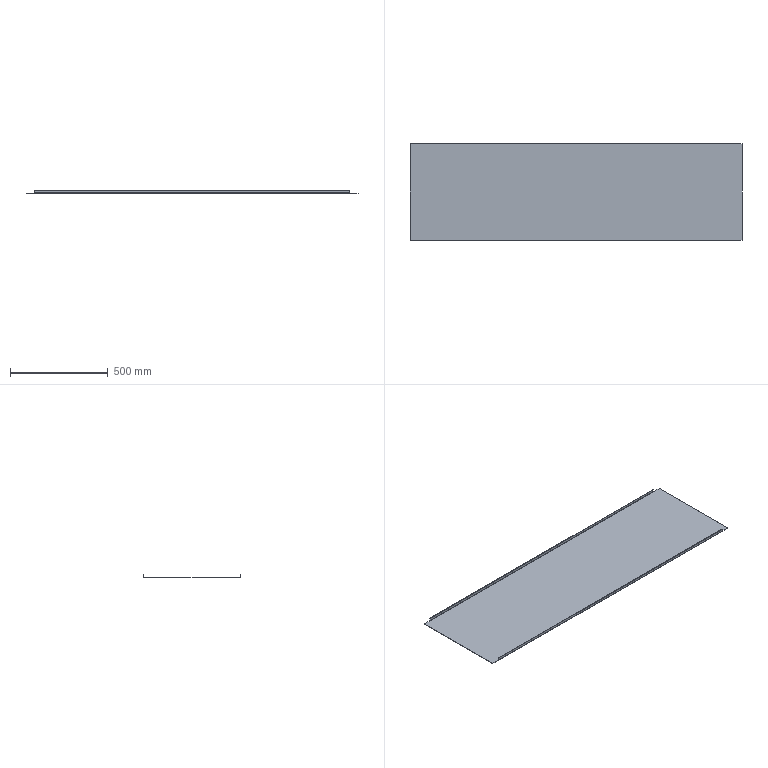Component | SolidWorks | RearBackPlate-1 | 1 solid | 22 faces | box 1700 x 500 x 15 mm | volume 1777475 mm3 | plane 18 | cylinder 4 | commonest cylinder face diameters 6 x2 2 x2
STEP:
#1=COLOUR_RGB('',0.7922,0.8196,0.9333);
#2=FILL_AREA_STYLE_COLOUR('',#1);
#3=FILL_AREA_STYLE('',(#2));
#4=SURFACE_STYLE_FILL_AREA(#3);
#5=SURFACE_SIDE_STYLE('',(#4));
#6=SURFACE_STYLE_USAGE(.BOTH.,#5);
#7=PRESENTATION_STYLE_ASSIGNMENT((#6));
#8=CARTESIAN_POINT('',(28.746,-4.158,0.03937));
#9=VERTEX_POINT('',#8);
#10=CARTESIAN_POINT('',(-34.876,-4.158,0.03937));
#11=VERTEX_POINT('',#10);
#12=CARTESIAN_POINT('',(-36.529,-4.158,0.03937));
#13=DIRECTION('',(-1.,0.,0.));
#14=VECTOR('',#13,39.37);
#15=LINE('',#12,#14);
#16=EDGE_CURVE('',#9,#11,#15,.T.);
#17=ORIENTED_EDGE('',*,*,#16,.T.);
#18=CARTESIAN_POINT('',(-34.876,-4.04,-0.07874));
#19=VERTEX_POINT('',#18);
#20=CARTESIAN_POINT('',(-34.876,-4.04,0.03937));
#21=DIRECTION('',(1.,0.,0.));
#22=DIRECTION('',(0.,0.,1.));
#23=AXIS2_PLACEMENT_3D('',#20,#21,#22);
#24=CIRCLE('',#23,0.1181);
#25=EDGE_CURVE('',#11,#19,#24,.T.);
#26=ORIENTED_EDGE('',*,*,#25,.T.);
#27=CARTESIAN_POINT('',(28.746,-4.04,-0.07874));
#28=VERTEX_POINT('',#27);
#29=CARTESIAN_POINT('',(30.4,-4.04,-0.07874));
#30=DIRECTION('',(-1.,0.,0.));
#31=VECTOR('',#30,39.37);
#32=LINE('',#29,#31);
#33=EDGE_CURVE('',#28,#19,#32,.T.);
#34=ORIENTED_EDGE('',*,*,#33,.F.);
#35=CARTESIAN_POINT('',(28.746,-4.04,0.03937));
#36=DIRECTION('',(1.,0.,0.));
#37=DIRECTION('',(0.,0.,1.));
#38=AXIS2_PLACEMENT_3D('',#35,#36,#37);
#39=CIRCLE('',#38,0.1181);
#40=EDGE_CURVE('',#9,#28,#39,.T.);
#41=ORIENTED_EDGE('',*,*,#40,.F.);
#42=EDGE_LOOP('',(#17,#26,#34,#41));
#43=FACE_OUTER_BOUND('',#42,.T.);
#44=CARTESIAN_POINT('',(30.4,-4.04,0.03937));
#45=DIRECTION('',(1.,0.,0.));
#46=DIRECTION('',(0.,-1.,-0.));
#47=AXIS2_PLACEMENT_3D('',#44,#45,#46);
#48=CYLINDRICAL_SURFACE('',#47,0.1181);
#49=ADVANCED_FACE('',(#43),#48,.T.);
#50=CARTESIAN_POINT('',(-34.876,-4.079,0.03937));
#51=VERTEX_POINT('',#50);
#52=CARTESIAN_POINT('',(-34.876,-4.04,-0.));
#53=VERTEX_POINT('',#52);
#54=CARTESIAN_POINT('',(-34.876,-4.04,0.03937));
#55=DIRECTION('',(1.,0.,0.));
#56=DIRECTION('',(0.,0.,1.));
#57=AXIS2_PLACEMENT_3D('',#54,#55,#56);
#58=CIRCLE('',#57,0.03937);
#59=EDGE_CURVE('',#51,#53,#58,.T.);
#60=ORIENTED_EDGE('',*,*,#59,.F.);
#61=CARTESIAN_POINT('',(28.746,-4.079,0.03937));
#62=VERTEX_POINT('',#61);
#63=CARTESIAN_POINT('',(-36.529,-4.079,0.03937));
#64=DIRECTION('',(1.,0.,0.));
#65=VECTOR('',#64,39.37);
#66=LINE('',#63,#65);
#67=EDGE_CURVE('',#51,#62,#66,.T.);
#68=ORIENTED_EDGE('',*,*,#67,.T.);
#69=CARTESIAN_POINT('',(28.746,-4.04,-0.));
#70=VERTEX_POINT('',#69);
#71=CARTESIAN_POINT('',(28.746,-4.04,0.03937));
#72=DIRECTION('',(1.,0.,0.));
#73=DIRECTION('',(0.,0.,1.));
#74=AXIS2_PLACEMENT_3D('',#71,#72,#73);
#75=CIRCLE('',#74,0.03937);
#76=EDGE_CURVE('',#62,#70,#75,.T.);
#77=ORIENTED_EDGE('',*,*,#76,.T.);
#78=CARTESIAN_POINT('',(30.4,-4.04,-0.));
#79=DIRECTION('',(-1.,0.,0.));
#80=VECTOR('',#79,39.37);
#81=LINE('',#78,#80);
#82=EDGE_CURVE('',#70,#53,#81,.T.);
#83=ORIENTED_EDGE('',*,*,#82,.T.);
#84=EDGE_LOOP('',(#60,#68,#77,#83));
#85=FACE_OUTER_BOUND('',#84,.T.);
#86=CARTESIAN_POINT('',(30.4,-4.04,0.03937));
#87=DIRECTION('',(1.,0.,0.));
#88=DIRECTION('',(0.,-1.,-0.));
#89=AXIS2_PLACEMENT_3D('',#86,#87,#88);
#90=CYLINDRICAL_SURFACE('',#89,0.03937);
#91=ADVANCED_FACE('',(#85),#90,.F.);
#92=CARTESIAN_POINT('',(-34.876,-4.158,0.5118));
#93=VERTEX_POINT('',#92);
#94=CARTESIAN_POINT('',(-34.876,-4.158,-0.07874));
#95=DIRECTION('',(0.,0.,1.));
#96=VECTOR('',#95,39.37);
#97=LINE('',#94,#96);
#98=EDGE_CURVE('',#11,#93,#97,.T.);
#99=ORIENTED_EDGE('',*,*,#98,.F.);
#100=ORIENTED_EDGE('',*,*,#16,.F.);
#101=CARTESIAN_POINT('',(28.746,-4.158,0.5118));
#102=VERTEX_POINT('',#101);
#103=CARTESIAN_POINT('',(28.746,-4.158,-0.07874));
#104=DIRECTION('',(0.,0.,-1.));
#105=VECTOR('',#104,39.37);
#106=LINE('',#103,#105);
#107=EDGE_CURVE('',#102,#9,#106,.T.);
#108=ORIENTED_EDGE('',*,*,#107,.F.);
#109=CARTESIAN_POINT('',(-36.529,-4.158,0.5118));
#110=DIRECTION('',(-1.,0.,0.));
#111=VECTOR('',#110,39.37);
#112=LINE('',#109,#111);
#113=EDGE_CURVE('',#102,#93,#112,.T.);
#114=ORIENTED_EDGE('',*,*,#113,.T.);
#115=EDGE_LOOP('',(#99,#100,#108,#114));
#116=FACE_OUTER_BOUND('',#115,.T.);
#117=CARTESIAN_POINT('',(-36.529,-4.158,0.5118));
#118=DIRECTION('',(0.,1.,0.));
#119=DIRECTION('',(0.,-0.,1.));
#120=AXIS2_PLACEMENT_3D('',#117,#118,#119);
#121=PLANE('',#120);
#122=ADVANCED_FACE('',(#116),#121,.F.);
#123=ORIENTED_EDGE('',*,*,#67,.F.);
#124=CARTESIAN_POINT('',(-34.876,-4.079,0.5118));
#125=VERTEX_POINT('',#124);
#126=CARTESIAN_POINT('',(-34.876,-4.079,0.5118));
#127=DIRECTION('',(0.,-0.,1.));
#128=VECTOR('',#127,39.37);
#129=LINE('',#126,#128);
#130=EDGE_CURVE('',#51,#125,#129,.T.);
#131=ORIENTED_EDGE('',*,*,#130,.T.);
#132=CARTESIAN_POINT('',(28.746,-4.079,0.5118));
#133=VERTEX_POINT('',#132);
#134=CARTESIAN_POINT('',(-36.529,-4.079,0.5118));
#135=DIRECTION('',(-1.,0.,0.));
#136=VECTOR('',#135,39.37);
#137=LINE('',#134,#136);
#138=EDGE_CURVE('',#133,#125,#137,.T.);
#139=ORIENTED_EDGE('',*,*,#138,.F.);
#140=CARTESIAN_POINT('',(28.746,-4.079,0.5118));
#141=DIRECTION('',(0.,-0.,1.));
#142=VECTOR('',#141,39.37);
#143=LINE('',#140,#142);
#144=EDGE_CURVE('',#62,#133,#143,.T.);
#145=ORIENTED_EDGE('',*,*,#144,.F.);
#146=EDGE_LOOP('',(#123,#131,#139,#145));
#147=FACE_OUTER_BOUND('',#146,.T.);
#148=CARTESIAN_POINT('',(-36.529,-4.079,0.5118));
#149=DIRECTION('',(0.,1.,0.));
#150=DIRECTION('',(0.,-0.,1.));
#151=AXIS2_PLACEMENT_3D('',#148,#149,#150);
#152=PLANE('',#151);
#153=ADVANCED_FACE('',(#147),#152,.T.);
#154=CARTESIAN_POINT('',(-34.876,-4.04,0.5118));
#155=DIRECTION('',(0.,1.,0.));
#156=VECTOR('',#155,39.37);
#157=LINE('',#154,#156);
#158=EDGE_CURVE('',#93,#125,#157,.T.);
#159=ORIENTED_EDGE('',*,*,#158,.F.);
#160=ORIENTED_EDGE('',*,*,#113,.F.);
#161=CARTESIAN_POINT('',(28.746,-4.158,0.5118));
#162=DIRECTION('',(0.,1.,0.));
#163=VECTOR('',#162,39.37);
#164=LINE('',#161,#163);
#165=EDGE_CURVE('',#102,#133,#164,.T.);
#166=ORIENTED_EDGE('',*,*,#165,.T.);
#167=ORIENTED_EDGE('',*,*,#138,.T.);
#168=EDGE_LOOP('',(#159,#160,#166,#167));
#169=FACE_OUTER_BOUND('',#168,.T.);
#170=CARTESIAN_POINT('',(-36.529,-4.158,0.5118));
#171=DIRECTION('',(0.,0.,-1.));
#172=DIRECTION('',(0.,1.,0.));
#173=AXIS2_PLACEMENT_3D('',#170,#171,#172);
#174=PLANE('',#173);
#175=ADVANCED_FACE('',(#169),#174,.F.);
#176=CARTESIAN_POINT('',(-34.876,15.527,0.03937));
#177=VERTEX_POINT('',#176);
#178=CARTESIAN_POINT('',(-34.876,15.409,-0.07874));
#179=VERTEX_POINT('',#178);
#180=CARTESIAN_POINT('',(-34.876,15.409,0.03937));
#181=DIRECTION('',(-1.,0.,0.));
#182=DIRECTION('',(0.,0.,-1.));
#183=AXIS2_PLACEMENT_3D('',#180,#181,#182);
#184=CIRCLE('',#183,0.1181);
#185=EDGE_CURVE('',#177,#179,#184,.T.);
#186=ORIENTED_EDGE('',*,*,#185,.F.);
#187=CARTESIAN_POINT('',(28.746,15.527,0.03937));
#188=VERTEX_POINT('',#187);
#189=CARTESIAN_POINT('',(30.4,15.527,0.03937));
#190=DIRECTION('',(1.,0.,0.));
#191=VECTOR('',#190,39.37);
#192=LINE('',#189,#191);
#193=EDGE_CURVE('',#177,#188,#192,.T.);
#194=ORIENTED_EDGE('',*,*,#193,.T.);
#195=CARTESIAN_POINT('',(28.746,15.409,-0.07874));
#196=VERTEX_POINT('',#195);
#197=CARTESIAN_POINT('',(28.746,15.409,0.03937));
#198=DIRECTION('',(-1.,0.,0.));
#199=DIRECTION('',(0.,-0.,-1.));
#200=AXIS2_PLACEMENT_3D('',#197,#198,#199);
#201=CIRCLE('',#200,0.1181);
#202=EDGE_CURVE('',#188,#196,#201,.T.);
#203=ORIENTED_EDGE('',*,*,#202,.T.);
#204=CARTESIAN_POINT('',(-36.529,15.409,-0.07874));
#205=DIRECTION('',(1.,0.,0.));
#206=VECTOR('',#205,39.37);
#207=LINE('',#204,#206);
#208=EDGE_CURVE('',#179,#196,#207,.T.);
#209=ORIENTED_EDGE('',*,*,#208,.F.);
#210=EDGE_LOOP('',(#186,#194,#203,#209));
#211=FACE_OUTER_BOUND('',#210,.T.);
#212=CARTESIAN_POINT('',(-36.529,15.409,0.03937));
#213=DIRECTION('',(-1.,0.,0.));
#214=DIRECTION('',(0.,1.,-0.));
#215=AXIS2_PLACEMENT_3D('',#212,#213,#214);
#216=CYLINDRICAL_SURFACE('',#215,0.1181);
#217=ADVANCED_FACE('',(#211),#216,.T.);
#218=CARTESIAN_POINT('',(28.746,15.449,0.03937));
#219=VERTEX_POINT('',#218);
#220=CARTESIAN_POINT('',(-34.876,15.449,0.03937));
#221=VERTEX_POINT('',#220);
#222=CARTESIAN_POINT('',(30.4,15.449,0.03937));
#223=DIRECTION('',(-1.,-0.,-0.));
#224=VECTOR('',#223,39.37);
#225=LINE('',#222,#224);
#226=EDGE_CURVE('',#219,#221,#225,.T.);
#227=ORIENTED_EDGE('',*,*,#226,.T.);
#228=CARTESIAN_POINT('',(-34.876,15.409,-0.));
#229=VERTEX_POINT('',#228);
#230=CARTESIAN_POINT('',(-34.876,15.409,0.03937));
#231=DIRECTION('',(-1.,0.,0.));
#232=DIRECTION('',(0.,0.,-1.));
#233=AXIS2_PLACEMENT_3D('',#230,#231,#232);
#234=CIRCLE('',#233,0.03937);
#235=EDGE_CURVE('',#221,#229,#234,.T.);
#236=ORIENTED_EDGE('',*,*,#235,.T.);
#237=CARTESIAN_POINT('',(28.746,15.409,-0.));
#238=VERTEX_POINT('',#237);
#239=CARTESIAN_POINT('',(-36.529,15.409,-0.));
#240=DIRECTION('',(1.,0.,0.));
#241=VECTOR('',#240,39.37);
#242=LINE('',#239,#241);
#243=EDGE_CURVE('',#229,#238,#242,.T.);
#244=ORIENTED_EDGE('',*,*,#243,.T.);
#245=CARTESIAN_POINT('',(28.746,15.409,0.03937));
#246=DIRECTION('',(-1.,0.,0.));
#247=DIRECTION('',(0.,-0.,-1.));
#248=AXIS2_PLACEMENT_3D('',#245,#246,#247);
#249=CIRCLE('',#248,0.03937);
#250=EDGE_CURVE('',#219,#238,#249,.T.);
#251=ORIENTED_EDGE('',*,*,#250,.F.);
#252=EDGE_LOOP('',(#227,#236,#244,#251));
#253=FACE_OUTER_BOUND('',#252,.T.);
#254=CARTESIAN_POINT('',(-36.529,15.409,0.03937));
#255=DIRECTION('',(-1.,0.,0.));
#256=DIRECTION('',(0.,1.,-0.));
#257=AXIS2_PLACEMENT_3D('',#254,#255,#256);
#258=CYLINDRICAL_SURFACE('',#257,0.03937);
#259=ADVANCED_FACE('',(#253),#258,.F.);
#260=ORIENTED_EDGE('',*,*,#193,.F.);
#261=CARTESIAN_POINT('',(-34.876,15.527,0.5118));
#262=VERTEX_POINT('',#261);
#263=CARTESIAN_POINT('',(-34.876,15.527,-0.07874));
#264=DIRECTION('',(0.,0.,-1.));
#265=VECTOR('',#264,39.37);
#266=LINE('',#263,#265);
#267=EDGE_CURVE('',#262,#177,#266,.T.);
#268=ORIENTED_EDGE('',*,*,#267,.F.);
#269=CARTESIAN_POINT('',(28.746,15.527,0.5118));
#270=VERTEX_POINT('',#269);
#271=CARTESIAN_POINT('',(30.4,15.527,0.5118));
#272=DIRECTION('',(1.,0.,0.));
#273=VECTOR('',#272,39.37);
#274=LINE('',#271,#273);
#275=EDGE_CURVE('',#262,#270,#274,.T.);
#276=ORIENTED_EDGE('',*,*,#275,.T.);
#277=CARTESIAN_POINT('',(28.746,15.527,-0.07874));
#278=DIRECTION('',(0.,0.,1.));
#279=VECTOR('',#278,39.37);
#280=LINE('',#277,#279);
#281=EDGE_CURVE('',#188,#270,#280,.T.);
#282=ORIENTED_EDGE('',*,*,#281,.F.);
#283=EDGE_LOOP('',(#260,#268,#276,#282));
#284=FACE_OUTER_BOUND('',#283,.T.);
#285=CARTESIAN_POINT('',(30.4,15.527,0.5118));
#286=DIRECTION('',(0.,-1.,0.));
#287=DIRECTION('',(0.,-0.,-1.));
#288=AXIS2_PLACEMENT_3D('',#285,#286,#287);
#289=PLANE('',#288);
#290=ADVANCED_FACE('',(#284),#289,.F.);
#291=CARTESIAN_POINT('',(-34.876,15.449,0.5118));
#292=VERTEX_POINT('',#291);
#293=CARTESIAN_POINT('',(-34.876,15.449,0.5118));
#294=DIRECTION('',(0.,0.,1.));
#295=VECTOR('',#294,39.37);
#296=LINE('',#293,#295);
#297=EDGE_CURVE('',#221,#292,#296,.T.);
#298=ORIENTED_EDGE('',*,*,#297,.F.);
#299=ORIENTED_EDGE('',*,*,#226,.F.);
#300=CARTESIAN_POINT('',(28.746,15.449,0.5118));
#301=VERTEX_POINT('',#300);
#302=CARTESIAN_POINT('',(28.746,15.449,0.5118));
#303=DIRECTION('',(0.,0.,1.));
#304=VECTOR('',#303,39.37);
#305=LINE('',#302,#304);
#306=EDGE_CURVE('',#219,#301,#305,.T.);
#307=ORIENTED_EDGE('',*,*,#306,.T.);
#308=CARTESIAN_POINT('',(30.4,15.449,0.5118));
#309=DIRECTION('',(1.,0.,0.));
#310=VECTOR('',#309,39.37);
#311=LINE('',#308,#310);
#312=EDGE_CURVE('',#292,#301,#311,.T.);
#313=ORIENTED_EDGE('',*,*,#312,.F.);
#314=EDGE_LOOP('',(#298,#299,#307,#313));
#315=FACE_OUTER_BOUND('',#314,.T.);
#316=CARTESIAN_POINT('',(30.4,15.449,0.5118));
#317=DIRECTION('',(0.,-1.,0.));
#318=DIRECTION('',(0.,-0.,-1.));
#319=AXIS2_PLACEMENT_3D('',#316,#317,#318);
#320=PLANE('',#319);
#321=ADVANCED_FACE('',(#315),#320,.T.);
#322=ORIENTED_EDGE('',*,*,#275,.F.);
#323=CARTESIAN_POINT('',(-34.876,15.409,0.5118));
#324=DIRECTION('',(0.,1.,0.));
#325=VECTOR('',#324,39.37);
#326=LINE('',#323,#325);
#327=EDGE_CURVE('',#292,#262,#326,.T.);
#328=ORIENTED_EDGE('',*,*,#327,.F.);
#329=ORIENTED_EDGE('',*,*,#312,.T.);
#330=CARTESIAN_POINT('',(28.746,15.409,0.5118));
#331=DIRECTION('',(0.,-1.,0.));
#332=VECTOR('',#331,39.37);
#333=LINE('',#330,#332);
#334=EDGE_CURVE('',#270,#301,#333,.T.);
#335=ORIENTED_EDGE('',*,*,#334,.F.);
#336=EDGE_LOOP('',(#322,#328,#329,#335));
#337=FACE_OUTER_BOUND('',#336,.T.);
#338=CARTESIAN_POINT('',(30.4,15.527,0.5118));
#339=DIRECTION('',(0.,-0.,-1.));
#340=DIRECTION('',(0.,1.,-0.));
#341=AXIS2_PLACEMENT_3D('',#338,#339,#340);
#342=PLANE('',#341);
#343=ADVANCED_FACE('',(#337),#342,.F.);
#344=CARTESIAN_POINT('',(-36.529,15.409,-0.07874));
#345=VERTEX_POINT('',#344);
#346=CARTESIAN_POINT('',(-36.529,15.409,-0.07874));
#347=DIRECTION('',(1.,0.,0.));
#348=VECTOR('',#347,39.37);
#349=LINE('',#346,#348);
#350=EDGE_CURVE('',#345,#179,#349,.T.);
#351=ORIENTED_EDGE('',*,*,#350,.T.);
#352=ORIENTED_EDGE('',*,*,#208,.T.);
#353=CARTESIAN_POINT('',(30.4,15.409,-0.07874));
#354=VERTEX_POINT('',#353);
#355=CARTESIAN_POINT('',(28.746,15.409,-0.07874));
#356=DIRECTION('',(1.,0.,0.));
#357=VECTOR('',#356,39.37);
#358=LINE('',#355,#357);
#359=EDGE_CURVE('',#196,#354,#358,.T.);
#360=ORIENTED_EDGE('',*,*,#359,.T.);
#361=CARTESIAN_POINT('',(30.4,-4.04,-0.07874));
#362=VERTEX_POINT('',#361);
#363=CARTESIAN_POINT('',(30.4,15.527,-0.07874));
#364=DIRECTION('',(0.,1.,0.));
#365=VECTOR('',#364,39.37);
#366=LINE('',#363,#365);
#367=EDGE_CURVE('',#362,#354,#366,.T.);
#368=ORIENTED_EDGE('',*,*,#367,.F.);
#369=CARTESIAN_POINT('',(30.4,-4.04,-0.07874));
#370=DIRECTION('',(-1.,0.,0.));
#371=VECTOR('',#370,39.37);
#372=LINE('',#369,#371);
#373=EDGE_CURVE('',#362,#28,#372,.T.);
#374=ORIENTED_EDGE('',*,*,#373,.T.);
#375=ORIENTED_EDGE('',*,*,#33,.T.);
#376=CARTESIAN_POINT('',(-36.529,-4.04,-0.07874));
#377=VERTEX_POINT('',#376);
#378=CARTESIAN_POINT('',(-34.876,-4.04,-0.07874));
#379=DIRECTION('',(-1.,0.,0.));
#380=VECTOR('',#379,39.37);
#381=LINE('',#378,#380);
#382=EDGE_CURVE('',#19,#377,#381,.T.);
#383=ORIENTED_EDGE('',*,*,#382,.T.);
#384=CARTESIAN_POINT('',(-36.529,15.527,-0.07874));
#385=DIRECTION('',(0.,-1.,0.));
#386=VECTOR('',#385,39.37);
#387=LINE('',#384,#386);
#388=EDGE_CURVE('',#345,#377,#387,.T.);
#389=ORIENTED_EDGE('',*,*,#388,.F.);
#390=EDGE_LOOP('',(#351,#352,#360,#368,#374,#375,#383,#389));
#391=FACE_OUTER_BOUND('',#390,.T.);
#392=CARTESIAN_POINT('',(30.4,-4.158,-0.07874));
#393=DIRECTION('',(0.,0.,1.));
#394=DIRECTION('',(1.,0.,0.));
#395=AXIS2_PLACEMENT_3D('',#392,#393,#394);
#396=PLANE('',#395);
#397=ADVANCED_FACE('',(#391),#396,.F.);
#398=CARTESIAN_POINT('',(30.4,-4.04,-0.));
#399=VERTEX_POINT('',#398);
#400=CARTESIAN_POINT('',(30.4,15.409,-0.));
#401=VERTEX_POINT('',#400);
#402=CARTESIAN_POINT('',(30.4,15.527,-0.));
#403=DIRECTION('',(0.,1.,0.));
#404=VECTOR('',#403,39.37);
#405=LINE('',#402,#404);
#406=EDGE_CURVE('',#399,#401,#405,.T.);
#407=ORIENTED_EDGE('',*,*,#406,.T.);
#408=CARTESIAN_POINT('',(-36.529,15.409,-0.));
#409=DIRECTION('',(1.,0.,0.));
#410=VECTOR('',#409,39.37);
#411=LINE('',#408,#410);
#412=EDGE_CURVE('',#238,#401,#411,.T.);
#413=ORIENTED_EDGE('',*,*,#412,.F.);
#414=ORIENTED_EDGE('',*,*,#243,.F.);
#415=CARTESIAN_POINT('',(-36.529,15.409,-0.));
#416=VERTEX_POINT('',#415);
#417=CARTESIAN_POINT('',(-36.529,15.409,-0.));
#418=DIRECTION('',(1.,0.,0.));
#419=VECTOR('',#418,39.37);
#420=LINE('',#417,#419);
#421=EDGE_CURVE('',#416,#229,#420,.T.);
#422=ORIENTED_EDGE('',*,*,#421,.F.);
#423=CARTESIAN_POINT('',(-36.529,-4.04,-0.));
#424=VERTEX_POINT('',#423);
#425=CARTESIAN_POINT('',(-36.529,15.527,-0.));
#426=DIRECTION('',(0.,-1.,0.));
#427=VECTOR('',#426,39.37);
#428=LINE('',#425,#427);
#429=EDGE_CURVE('',#416,#424,#428,.T.);
#430=ORIENTED_EDGE('',*,*,#429,.T.);
#431=CARTESIAN_POINT('',(30.4,-4.04,-0.));
#432=DIRECTION('',(-1.,0.,0.));
#433=VECTOR('',#432,39.37);
#434=LINE('',#431,#433);
#435=EDGE_CURVE('',#53,#424,#434,.T.);
#436=ORIENTED_EDGE('',*,*,#435,.F.);
#437=ORIENTED_EDGE('',*,*,#82,.F.);
#438=CARTESIAN_POINT('',(30.4,-4.04,-0.));
#439=DIRECTION('',(-1.,0.,0.));
#440=VECTOR('',#439,39.37);
#441=LINE('',#438,#440);
#442=EDGE_CURVE('',#399,#70,#441,.T.);
#443=ORIENTED_EDGE('',*,*,#442,.F.);
#444=EDGE_LOOP('',(#407,#413,#414,#422,#430,#436,#437,#443));
#445=FACE_OUTER_BOUND('',#444,.T.);
#446=CARTESIAN_POINT('',(30.4,-4.158,-0.));
#447=DIRECTION('',(0.,0.,1.));
#448=DIRECTION('',(1.,0.,0.));
#449=AXIS2_PLACEMENT_3D('',#446,#447,#448);
#450=PLANE('',#449);
#451=ADVANCED_FACE('',(#445),#450,.T.);
#452=ORIENTED_EDGE('',*,*,#429,.F.);
#453=CARTESIAN_POINT('',(-36.529,15.409,-0.));
#454=DIRECTION('',(0.,0.,-1.));
#455=VECTOR('',#454,39.37);
#456=LINE('',#453,#455);
#457=EDGE_CURVE('',#416,#345,#456,.T.);
#458=ORIENTED_EDGE('',*,*,#457,.T.);
#459=ORIENTED_EDGE('',*,*,#388,.T.);
#460=CARTESIAN_POINT('',(-36.529,-4.04,-0.));
#461=DIRECTION('',(0.,0.,-1.));
#462=VECTOR('',#461,39.37);
#463=LINE('',#460,#462);
#464=EDGE_CURVE('',#424,#377,#463,.T.);
#465=ORIENTED_EDGE('',*,*,#464,.F.);
#466=EDGE_LOOP('',(#452,#458,#459,#465));
#467=FACE_OUTER_BOUND('',#466,.T.);
#468=CARTESIAN_POINT('',(-36.529,15.527,-0.07874));
#469=DIRECTION('',(-1.,-0.,0.));
#470=DIRECTION('',(0.,-1.,0.));
#471=AXIS2_PLACEMENT_3D('',#468,#469,#470);
#472=PLANE('',#471);
#473=ADVANCED_FACE('',(#467),#472,.T.);
#474=CARTESIAN_POINT('',(30.4,15.409,-0.));
#475=DIRECTION('',(0.,0.,-1.));
#476=VECTOR('',#475,39.37);
#477=LINE('',#474,#476);
#478=EDGE_CURVE('',#401,#354,#477,.T.);
#479=ORIENTED_EDGE('',*,*,#478,.F.);
#480=ORIENTED_EDGE('',*,*,#406,.F.);
#481=CARTESIAN_POINT('',(30.4,-4.04,-0.));
#482=DIRECTION('',(0.,0.,-1.));
#483=VECTOR('',#482,39.37);
#484=LINE('',#481,#483);
#485=EDGE_CURVE('',#399,#362,#484,.T.);
#486=ORIENTED_EDGE('',*,*,#485,.T.);
#487=ORIENTED_EDGE('',*,*,#367,.T.);
#488=EDGE_LOOP('',(#479,#480,#486,#487));
#489=FACE_OUTER_BOUND('',#488,.T.);
#490=CARTESIAN_POINT('',(30.4,15.527,-0.07874));
#491=DIRECTION('',(1.,-0.,0.));
#492=DIRECTION('',(0.,1.,0.));
#493=AXIS2_PLACEMENT_3D('',#490,#491,#492);
#494=PLANE('',#493);
#495=ADVANCED_FACE('',(#489),#494,.T.);
#496=CARTESIAN_POINT('',(28.746,-4.04,-0.07874));
#497=DIRECTION('',(0.,0.,1.));
#498=VECTOR('',#497,39.37);
#499=LINE('',#496,#498);
#500=EDGE_CURVE('',#28,#70,#499,.T.);
#501=ORIENTED_EDGE('',*,*,#500,.F.);
#502=ORIENTED_EDGE('',*,*,#373,.F.);
#503=ORIENTED_EDGE('',*,*,#485,.F.);
#504=ORIENTED_EDGE('',*,*,#442,.T.);
#505=EDGE_LOOP('',(#501,#502,#503,#504));
#506=FACE_OUTER_BOUND('',#505,.T.);
#507=CARTESIAN_POINT('',(28.746,-4.04,-0.07874));
#508=DIRECTION('',(0.,1.,0.));
#509=DIRECTION('',(0.,0.,1.));
#510=AXIS2_PLACEMENT_3D('',#507,#508,#509);
#511=PLANE('',#510);
#512=ADVANCED_FACE('',(#506),#511,.F.);
#513=ORIENTED_EDGE('',*,*,#40,.T.);
#514=ORIENTED_EDGE('',*,*,#500,.T.);
#515=ORIENTED_EDGE('',*,*,#76,.F.);
#516=ORIENTED_EDGE('',*,*,#144,.T.);
#517=ORIENTED_EDGE('',*,*,#165,.F.);
#518=ORIENTED_EDGE('',*,*,#107,.T.);
#519=EDGE_LOOP('',(#513,#514,#515,#516,#517,#518));
#520=FACE_OUTER_BOUND('',#519,.T.);
#521=CARTESIAN_POINT('',(28.746,-4.158,-0.07874));
#522=DIRECTION('',(-1.,0.,0.));
#523=DIRECTION('',(0.,0.,1.));
#524=AXIS2_PLACEMENT_3D('',#521,#522,#523);
#525=PLANE('',#524);
#526=ADVANCED_FACE('',(#520),#525,.F.);
#527=ORIENTED_EDGE('',*,*,#478,.T.);
#528=ORIENTED_EDGE('',*,*,#359,.F.);
#529=CARTESIAN_POINT('',(28.746,15.409,-0.07874));
#530=DIRECTION('',(0.,0.,-1.));
#531=VECTOR('',#530,39.37);
#532=LINE('',#529,#531);
#533=EDGE_CURVE('',#238,#196,#532,.T.);
#534=ORIENTED_EDGE('',*,*,#533,.F.);
#535=ORIENTED_EDGE('',*,*,#412,.T.);
#536=EDGE_LOOP('',(#527,#528,#534,#535));
#537=FACE_OUTER_BOUND('',#536,.T.);
#538=CARTESIAN_POINT('',(28.746,15.409,-0.07874));
#539=DIRECTION('',(0.,-1.,0.));
#540=DIRECTION('',(0.,0.,-1.));
#541=AXIS2_PLACEMENT_3D('',#538,#539,#540);
#542=PLANE('',#541);
#543=ADVANCED_FACE('',(#537),#542,.F.);
#544=ORIENTED_EDGE('',*,*,#281,.T.);
#545=ORIENTED_EDGE('',*,*,#334,.T.);
#546=ORIENTED_EDGE('',*,*,#306,.F.);
#547=ORIENTED_EDGE('',*,*,#250,.T.);
#548=ORIENTED_EDGE('',*,*,#533,.T.);
#549=ORIENTED_EDGE('',*,*,#202,.F.);
#550=EDGE_LOOP('',(#544,#545,#546,#547,#548,#549));
#551=FACE_OUTER_BOUND('',#550,.T.);
#552=CARTESIAN_POINT('',(28.746,15.527,-0.07874));
#553=DIRECTION('',(1.,0.,0.));
#554=DIRECTION('',(0.,0.,-1.));
#555=AXIS2_PLACEMENT_3D('',#552,#553,#554);
#556=PLANE('',#555);
#557=ADVANCED_FACE('',(#551),#556,.T.);
#558=ORIENTED_EDGE('',*,*,#185,.T.);
#559=CARTESIAN_POINT('',(-34.876,15.409,-0.07874));
#560=DIRECTION('',(0.,0.,1.));
#561=VECTOR('',#560,39.37);
#562=LINE('',#559,#561);
#563=EDGE_CURVE('',#179,#229,#562,.T.);
#564=ORIENTED_EDGE('',*,*,#563,.T.);
#565=ORIENTED_EDGE('',*,*,#235,.F.);
#566=ORIENTED_EDGE('',*,*,#297,.T.);
#567=ORIENTED_EDGE('',*,*,#327,.T.);
#568=ORIENTED_EDGE('',*,*,#267,.T.);
#569=EDGE_LOOP('',(#558,#564,#565,#566,#567,#568));
#570=FACE_OUTER_BOUND('',#569,.T.);
#571=CARTESIAN_POINT('',(-34.876,15.527,-0.07874));
#572=DIRECTION('',(1.,0.,0.));
#573=DIRECTION('',(0.,0.,-1.));
#574=AXIS2_PLACEMENT_3D('',#571,#572,#573);
#575=PLANE('',#574);
#576=ADVANCED_FACE('',(#570),#575,.F.);
#577=ORIENTED_EDGE('',*,*,#421,.T.);
#578=ORIENTED_EDGE('',*,*,#563,.F.);
#579=ORIENTED_EDGE('',*,*,#350,.F.);
#580=ORIENTED_EDGE('',*,*,#457,.F.);
#581=EDGE_LOOP('',(#577,#578,#579,#580));
#582=FACE_OUTER_BOUND('',#581,.T.);
#583=CARTESIAN_POINT('',(-34.876,15.409,-0.07874));
#584=DIRECTION('',(0.,-1.,0.));
#585=DIRECTION('',(0.,0.,-1.));
#586=AXIS2_PLACEMENT_3D('',#583,#584,#585);
#587=PLANE('',#586);
#588=ADVANCED_FACE('',(#582),#587,.F.);
#589=ORIENTED_EDGE('',*,*,#464,.T.);
#590=ORIENTED_EDGE('',*,*,#382,.F.);
#591=CARTESIAN_POINT('',(-34.876,-4.04,-0.07874));
#592=DIRECTION('',(0.,0.,-1.));
#593=VECTOR('',#592,39.37);
#594=LINE('',#591,#593);
#595=EDGE_CURVE('',#53,#19,#594,.T.);
#596=ORIENTED_EDGE('',*,*,#595,.F.);
#597=ORIENTED_EDGE('',*,*,#435,.T.);
#598=EDGE_LOOP('',(#589,#590,#596,#597));
#599=FACE_OUTER_BOUND('',#598,.T.);
#600=CARTESIAN_POINT('',(-34.876,-4.04,-0.07874));
#601=DIRECTION('',(0.,1.,0.));
#602=DIRECTION('',(0.,0.,1.));
#603=AXIS2_PLACEMENT_3D('',#600,#601,#602);
#604=PLANE('',#603);
#605=ADVANCED_FACE('',(#599),#604,.F.);
#606=ORIENTED_EDGE('',*,*,#98,.T.);
#607=ORIENTED_EDGE('',*,*,#158,.T.);
#608=ORIENTED_EDGE('',*,*,#130,.F.);
#609=ORIENTED_EDGE('',*,*,#59,.T.);
#610=ORIENTED_EDGE('',*,*,#595,.T.);
#611=ORIENTED_EDGE('',*,*,#25,.F.);
#612=EDGE_LOOP('',(#606,#607,#608,#609,#610,#611));
#613=FACE_OUTER_BOUND('',#612,.T.);
#614=CARTESIAN_POINT('',(-34.876,-4.158,-0.07874));
#615=DIRECTION('',(-1.,0.,0.));
#616=DIRECTION('',(0.,0.,1.));
#617=AXIS2_PLACEMENT_3D('',#614,#615,#616);
#618=PLANE('',#617);
#619=ADVANCED_FACE('',(#613),#618,.T.);
#620=CLOSED_SHELL('',(#49,#91,#122,#153,#175,#217,#259,#290,#321,#343,#397,#451,#473,#495,#512,#526,#543,#557,#576,#588,#605,#619));
#621=MANIFOLD_SOLID_BREP('',#620);
#622=STYLED_ITEM('',(#7),#621);
#623=PRESENTATION_LAYER_ASSIGNMENT('','',(#622));
#624=(LENGTH_UNIT()NAMED_UNIT(*)SI_UNIT($,.METRE.));
#625=LENGTH_MEASURE_WITH_UNIT(LENGTH_MEASURE(0.0254),#624);
#626=DIMENSIONAL_EXPONENTS(1.,0.,0.,0.,0.,0.,0.);
#627=(CONVERSION_BASED_UNIT('',#625)LENGTH_UNIT()NAMED_UNIT(#626));
#628=UNCERTAINTY_MEASURE_WITH_UNIT(LENGTH_MEASURE(0.00001),#627,'','');
#629=(NAMED_UNIT(*)PLANE_ANGLE_UNIT()SI_UNIT($,.RADIAN.));
#630=(NAMED_UNIT(*)SI_UNIT($,.STERADIAN.)SOLID_ANGLE_UNIT());
#631=(GEOMETRIC_REPRESENTATION_CONTEXT(3)GLOBAL_UNCERTAINTY_ASSIGNED_CONTEXT((#628))GLOBAL_UNIT_ASSIGNED_CONTEXT((#627,#629,#630))REPRESENTATION_CONTEXT('',''));
#632=MECHANICAL_DESIGN_GEOMETRIC_PRESENTATION_REPRESENTATION('',(#622),#631);
#633=CARTESIAN_POINT('',(0.,0.,0.));
#634=DIRECTION('',(0.,0.,1.));
#635=DIRECTION('',(1.,0.,0.));
#636=AXIS2_PLACEMENT_3D('',#633,#634,#635);
#637=(LENGTH_UNIT()NAMED_UNIT(*)SI_UNIT($,.METRE.));
#638=LENGTH_MEASURE_WITH_UNIT(LENGTH_MEASURE(0.0254),#637);
#639=DIMENSIONAL_EXPONENTS(1.,0.,0.,0.,0.,0.,0.);
#640=(CONVERSION_BASED_UNIT('',#638)LENGTH_UNIT()NAMED_UNIT(#639));
#641=UNCERTAINTY_MEASURE_WITH_UNIT(LENGTH_MEASURE(0.00001),#640,'','');
#642=(NAMED_UNIT(*)PLANE_ANGLE_UNIT()SI_UNIT($,.RADIAN.));
#643=(NAMED_UNIT(*)SI_UNIT($,.STERADIAN.)SOLID_ANGLE_UNIT());
#644=(GEOMETRIC_REPRESENTATION_CONTEXT(3)GLOBAL_UNCERTAINTY_ASSIGNED_CONTEXT((#641))GLOBAL_UNIT_ASSIGNED_CONTEXT((#640,#642,#643))REPRESENTATION_CONTEXT('',''));
#645=ADVANCED_BREP_SHAPE_REPRESENTATION('',(#621,#636),#644);